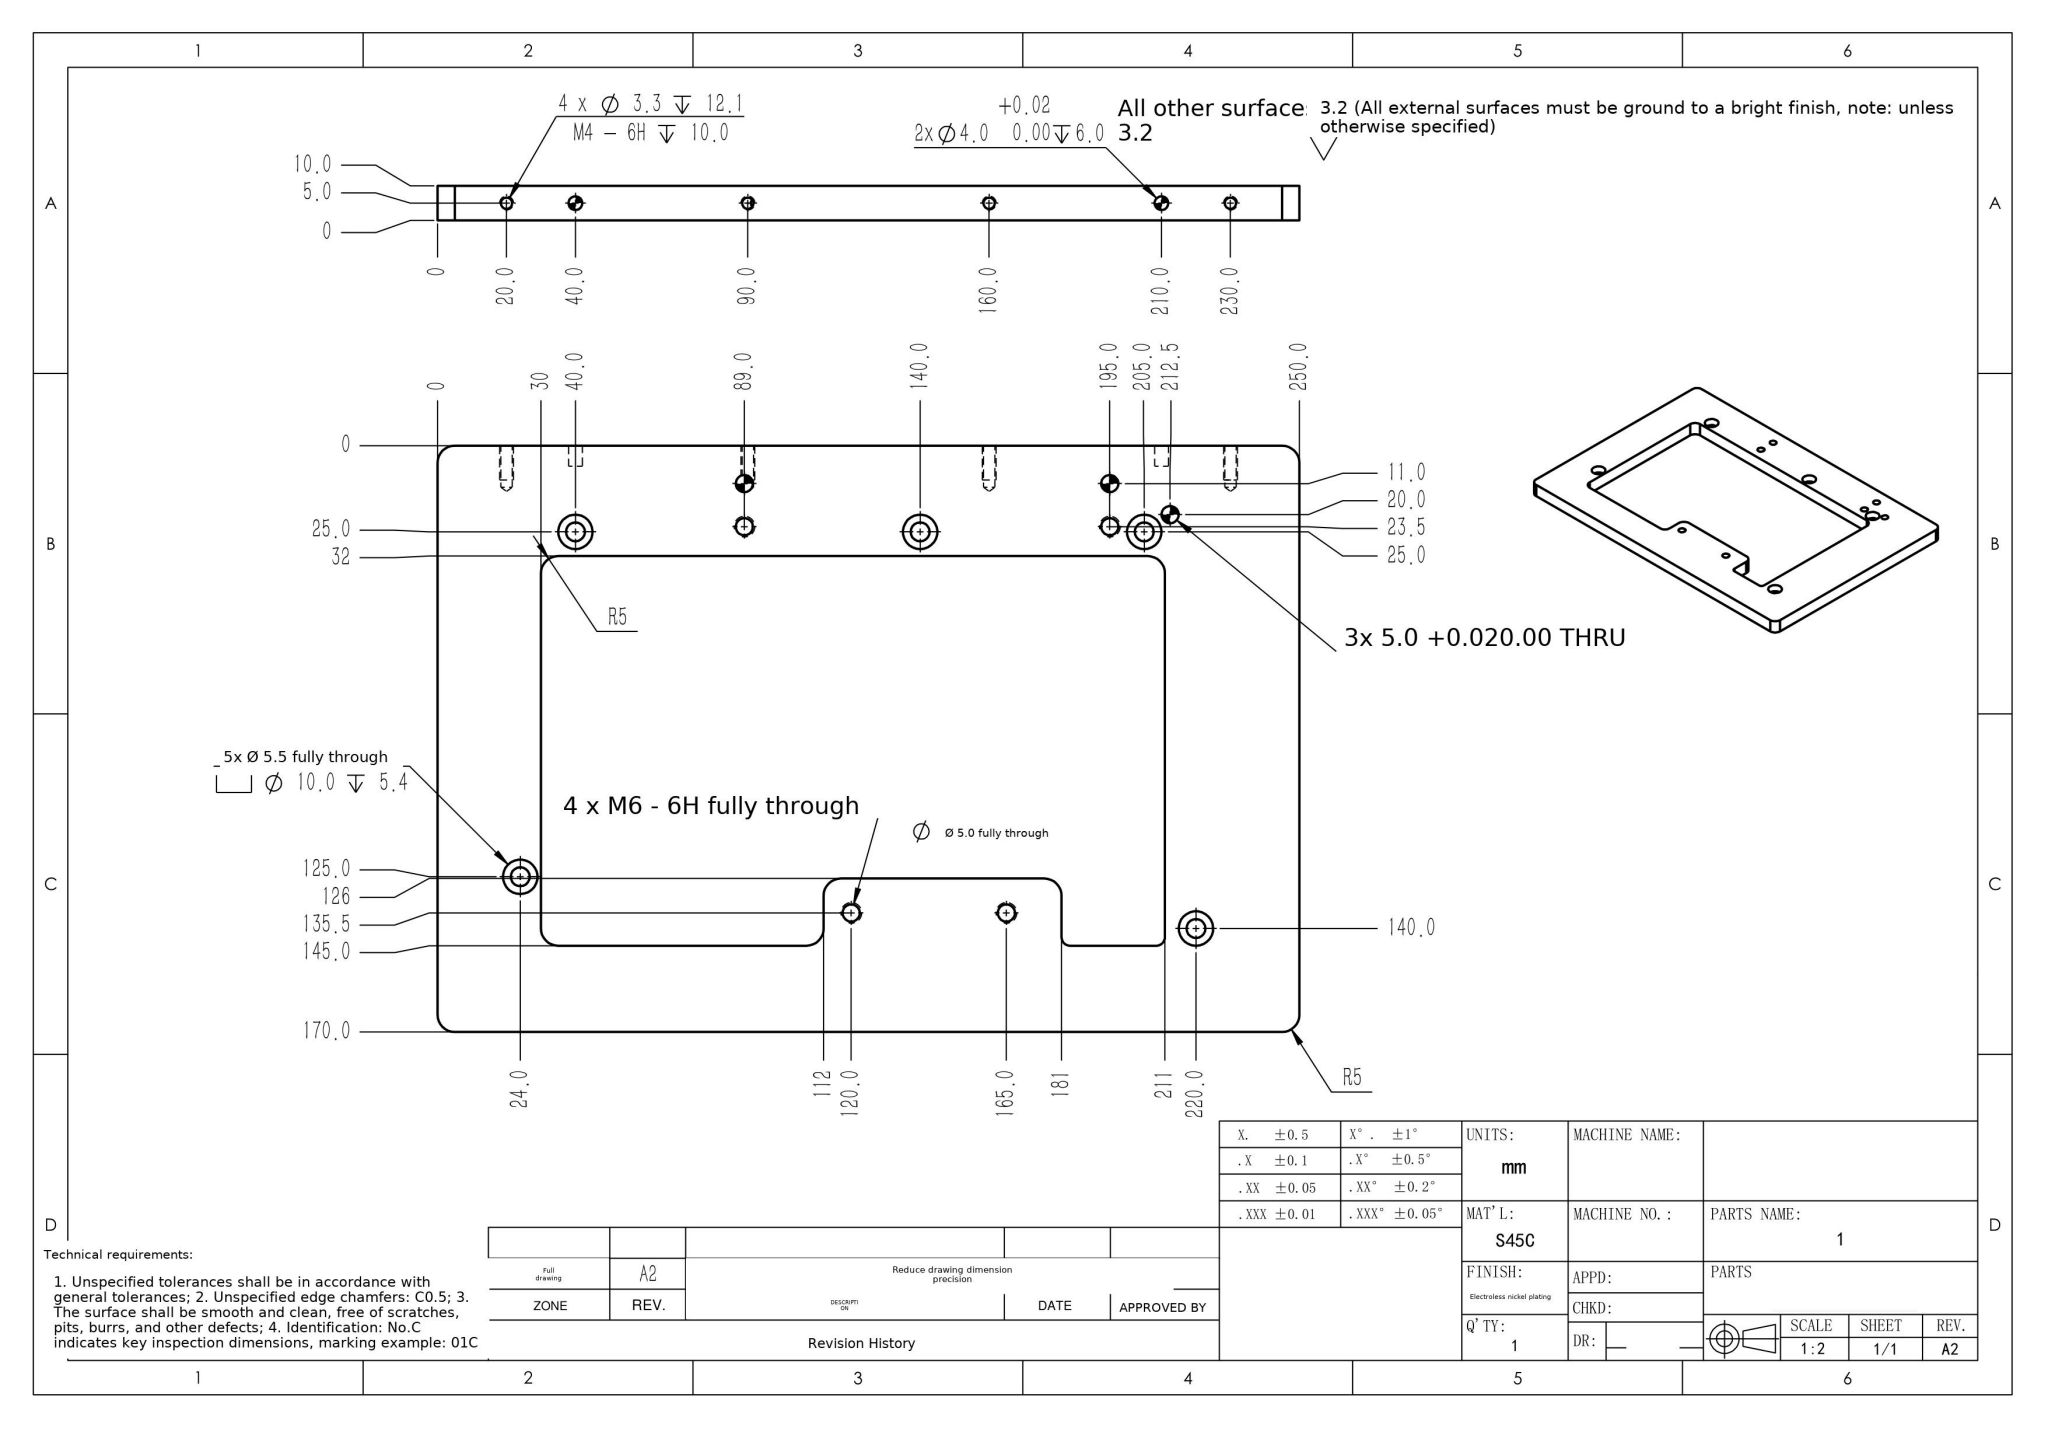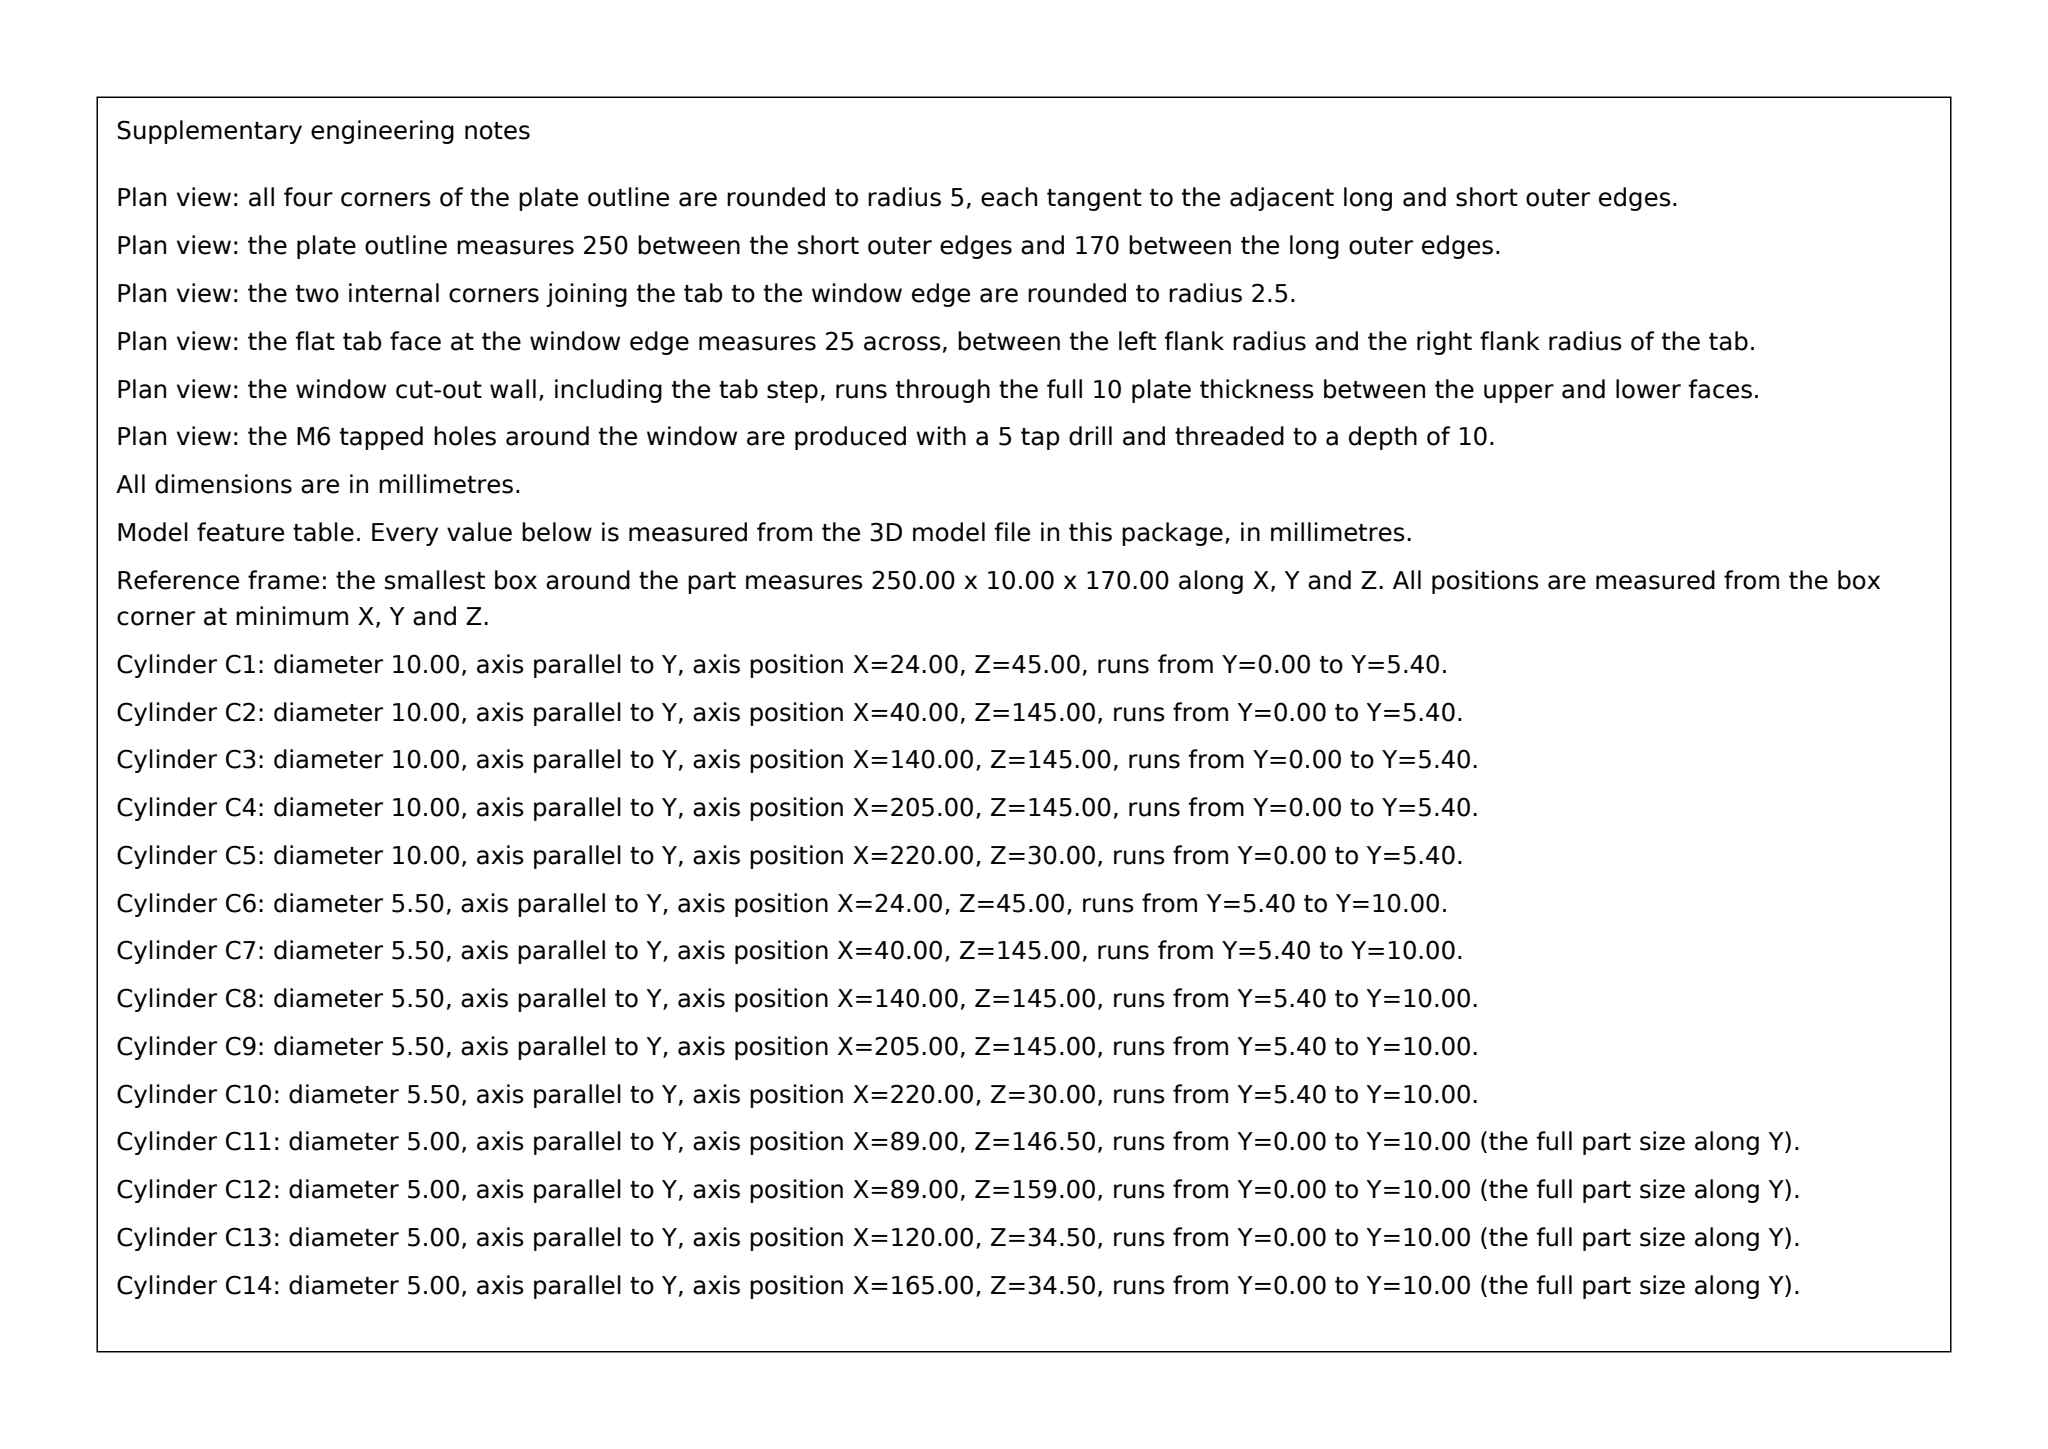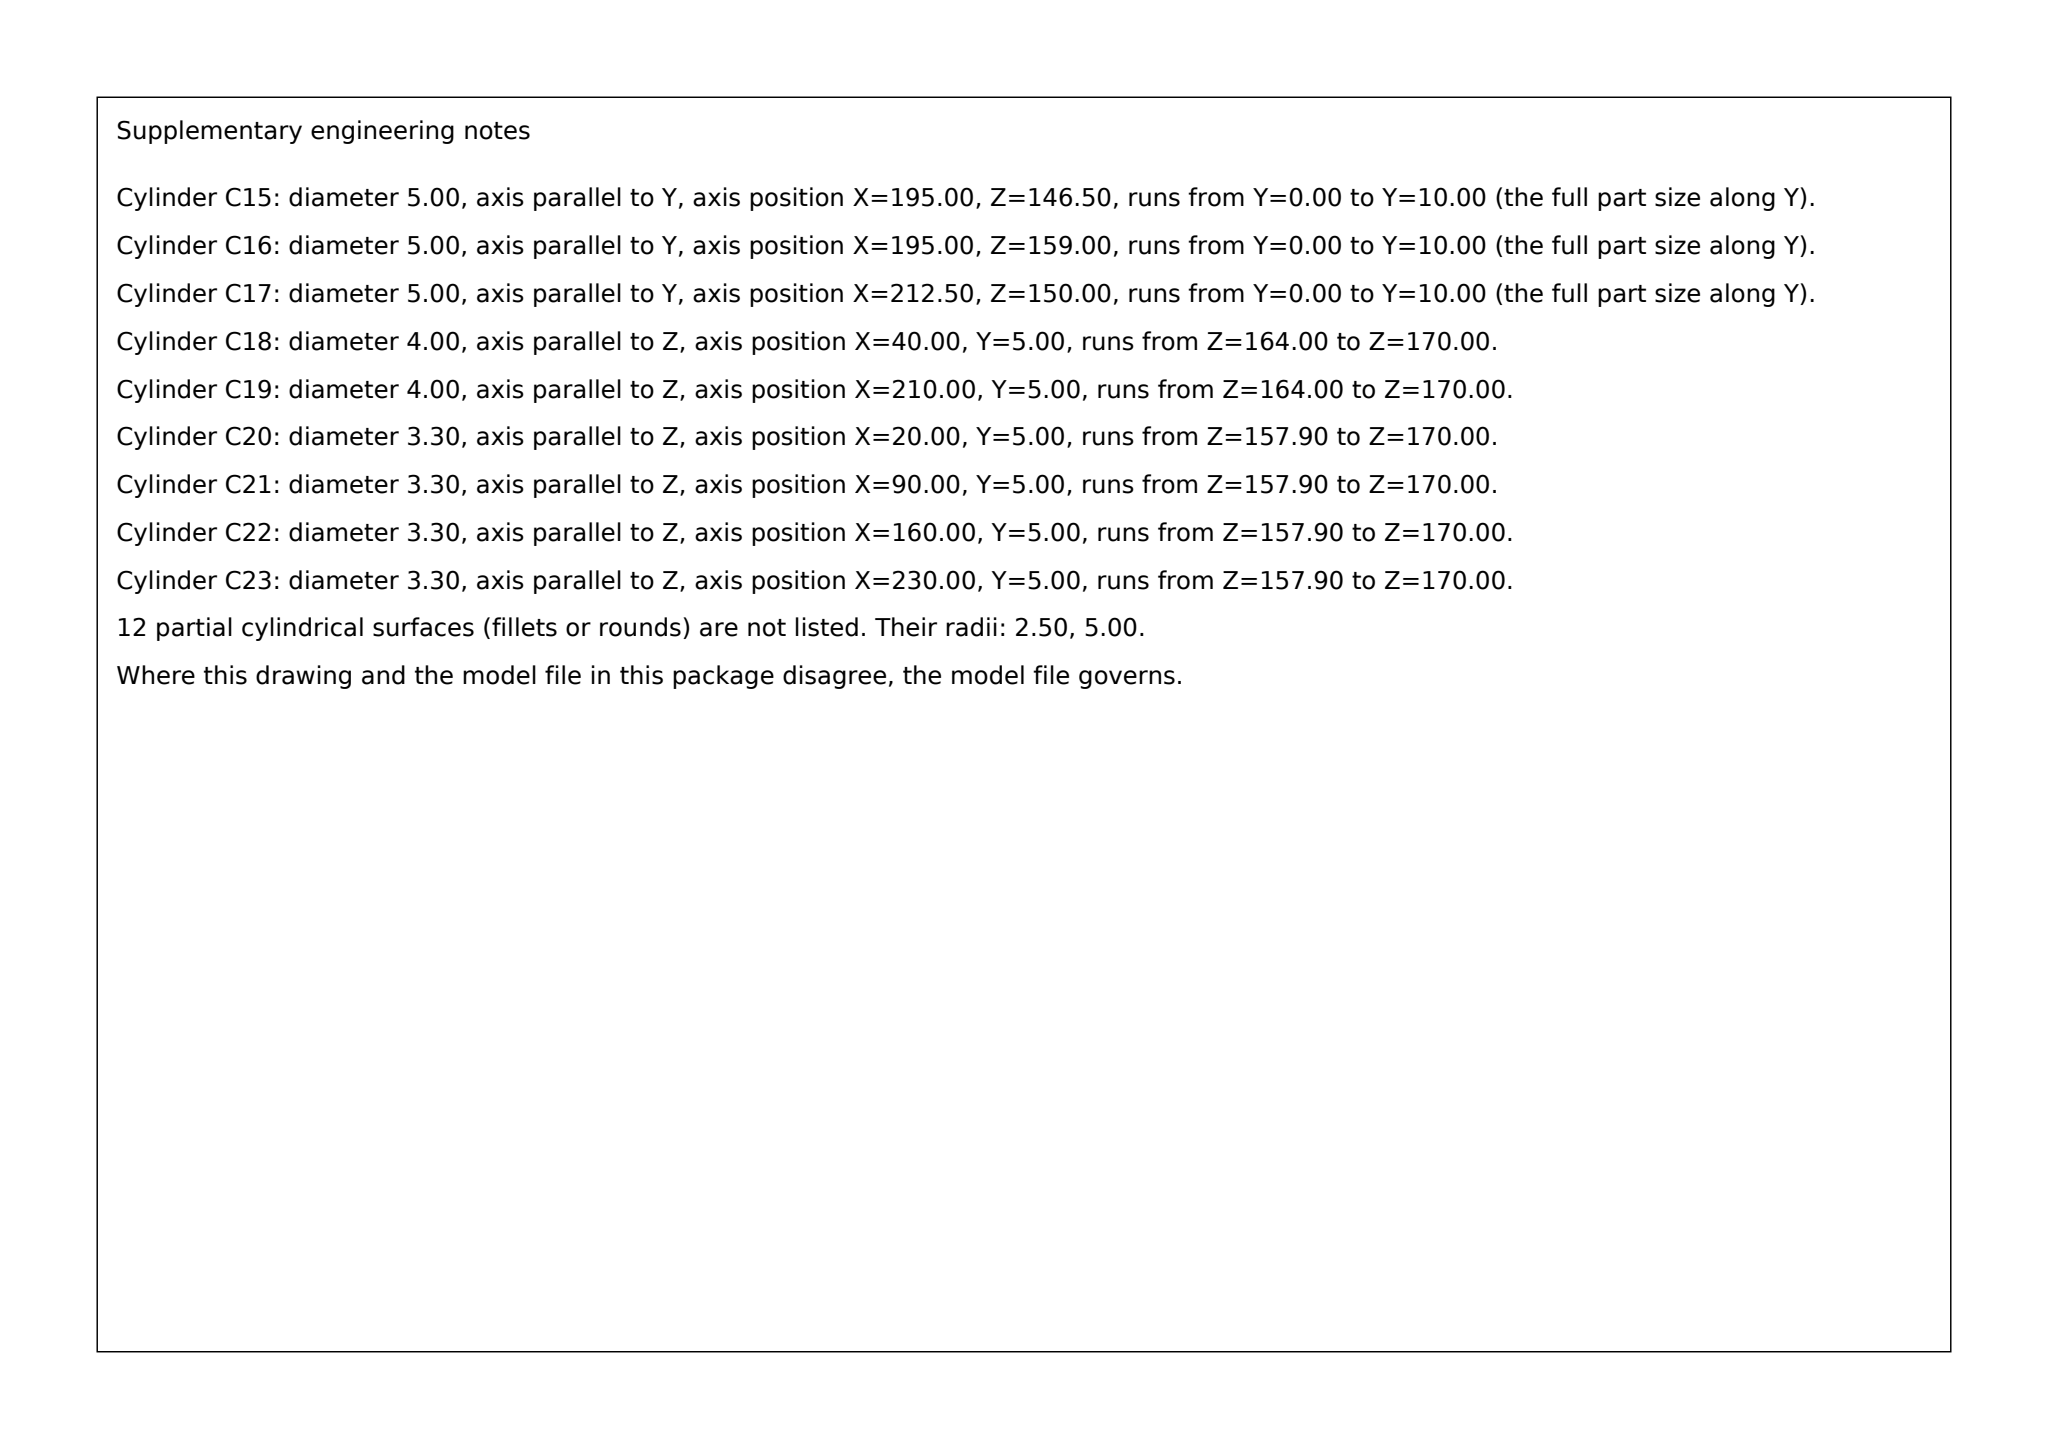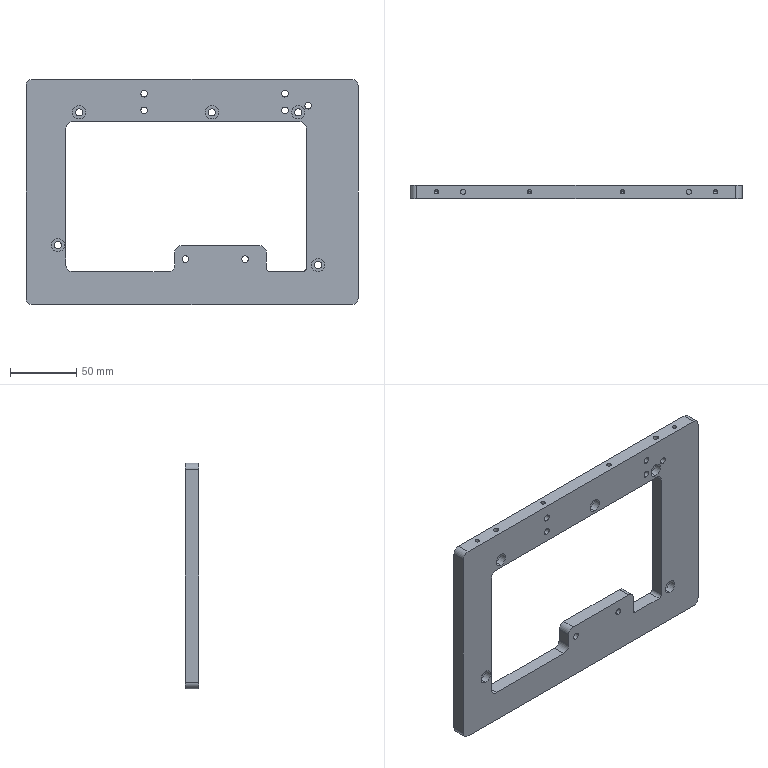Part | SolidWorks | mm | 1 solid | 89 faces | box 250 x 10 x 170 mm | volume 229255 mm3 | cylinder 58 | plane 21 | cone 10 | commonest cylinder face diameters 10 x20 5 x16 5.5 x10 3.3 x8 4 x4
Drawing notes:
R5 TYP: 4X OUTER CORNERS, 6X CUT-OUT CORNERS INCL STEPS AT X=112 & 181 | from the solid: Ø10 y-axis cyls L=10 at (5,5),(5,165),(245,5),(245,165) outer; (35,30),(35,133),(107,30),(206,133),(117,39.5),(176,39.5) cut-out, tangent to x=112/x=181 and z=44.5
5X Ø5.5 THRU with C'BORE Ø10.0 ▼5.4 MACHINED FROM THE Y=0 FACE ONLY (counterbore opens on that face; opposite face Y=10 is plain). | from the solid: cylinders Ø10.0 axis y from 0.0 to 5.4 paired with Ø5.5 axis y from 5.4 to 10.0 at the same 5 centres; axis_planes y=5.4 counterbore bottoms
2X R5 external round at the cut-out step, arc centres X=117 and X=176, 130.5 from top datum. | from the solid: convex arc (round/outer radius) dia 10.0 axis y at [117,null,39.5] and [176,null,39.5] (170-39.5 = 130.5)
2X R2.5 internal fillets at the lower cut-out recess, arc centres X=183.5 and X=208.5, 142.5 from top datum. | from the solid: concave arc dia 5.0, axis y at [183.5,27.5] and [208.5,27.5], 90 deg